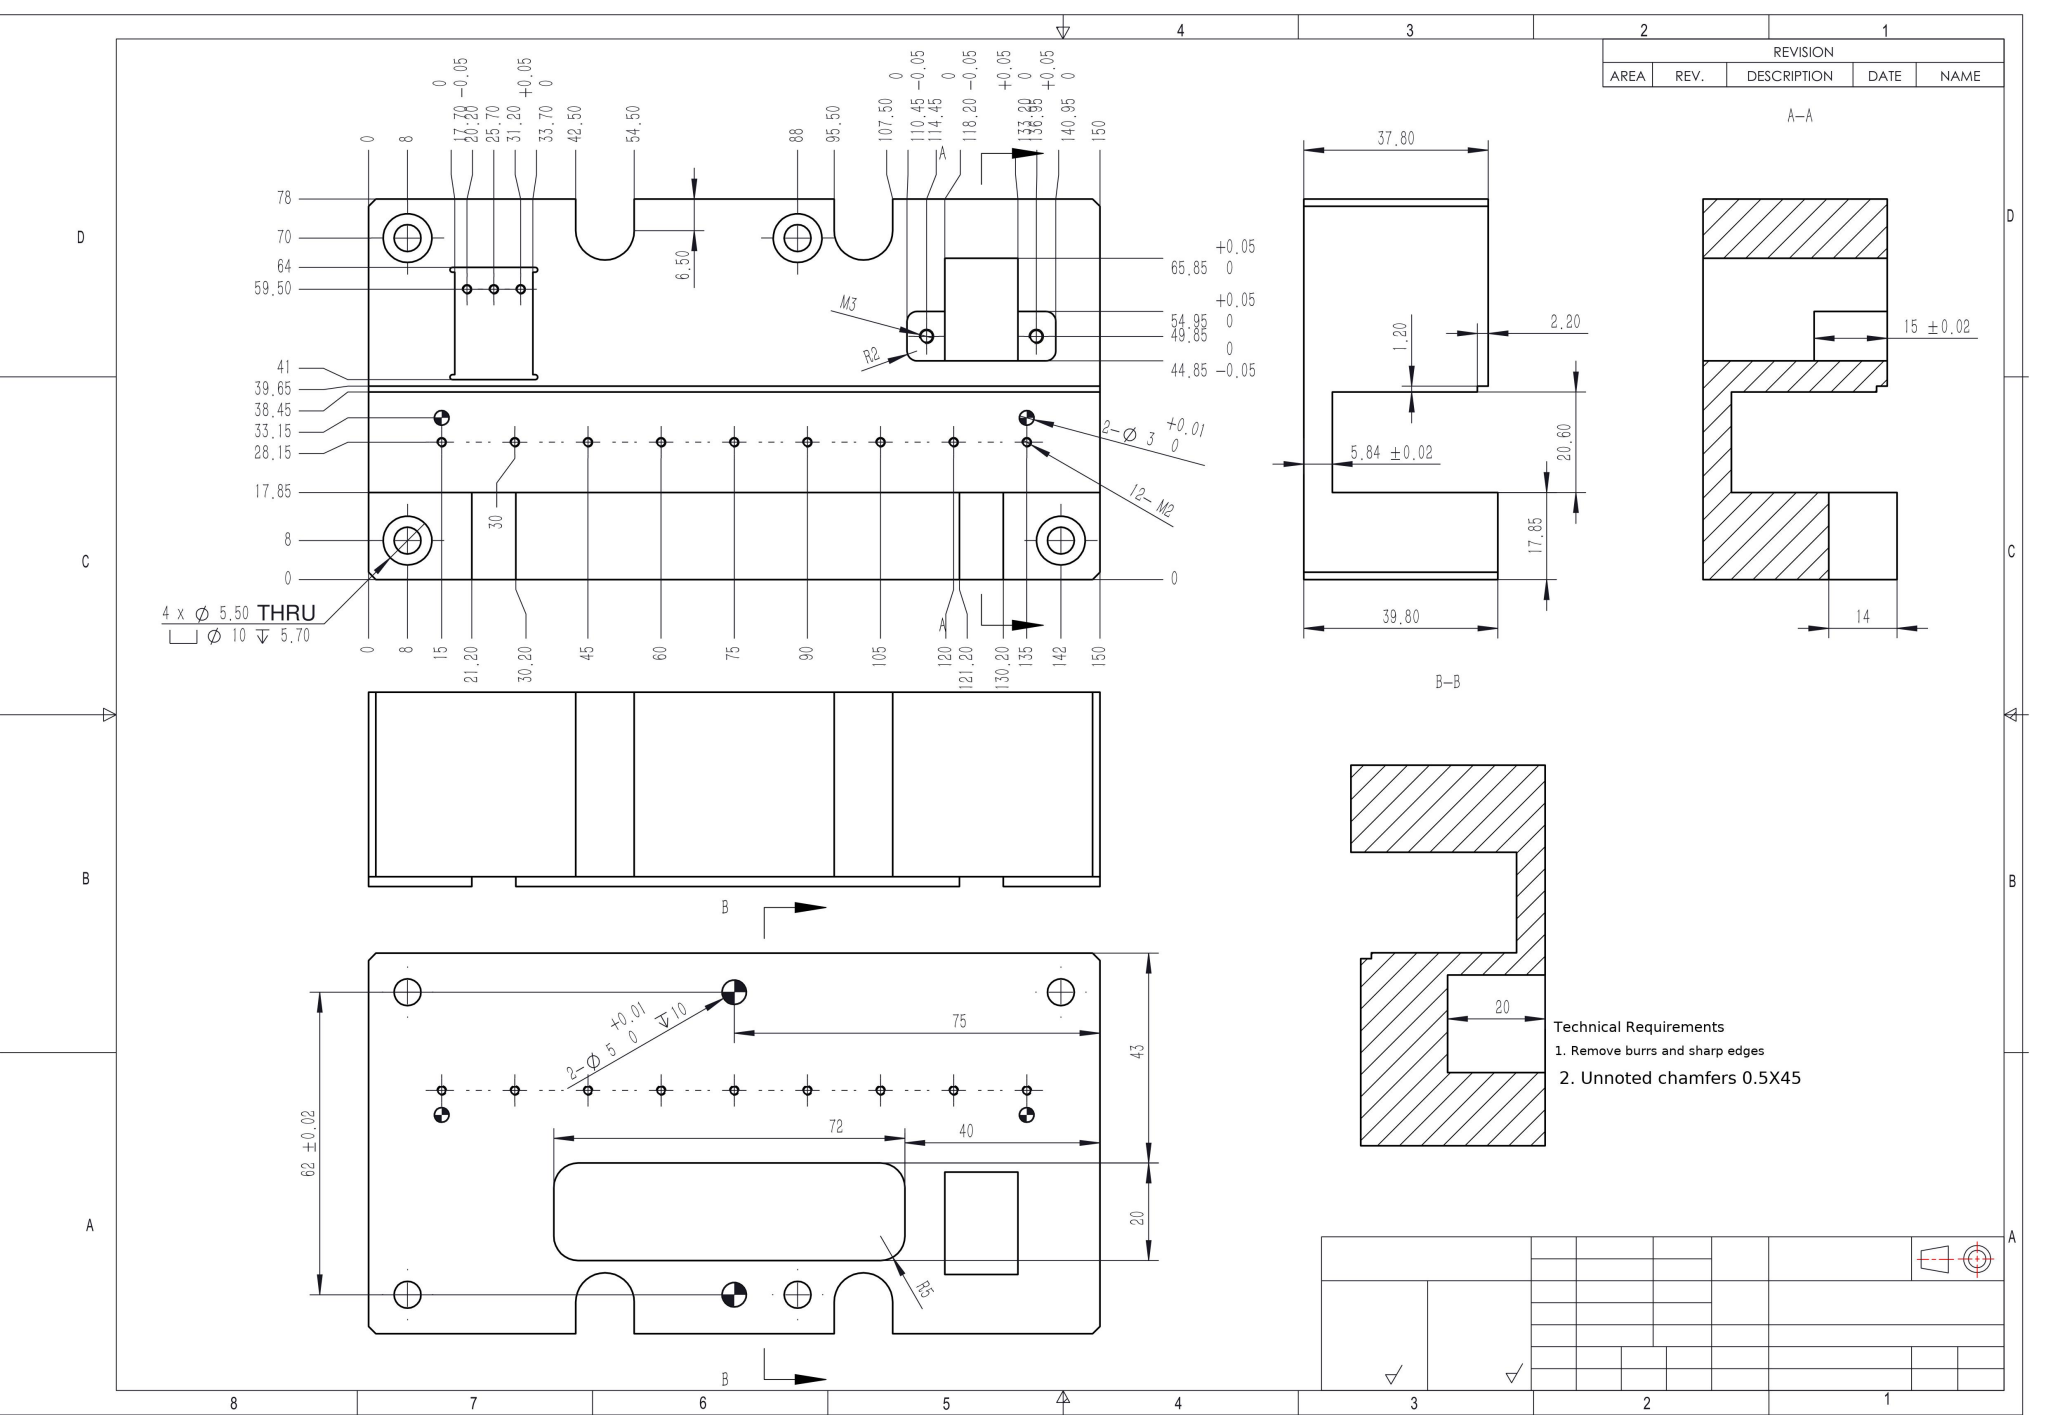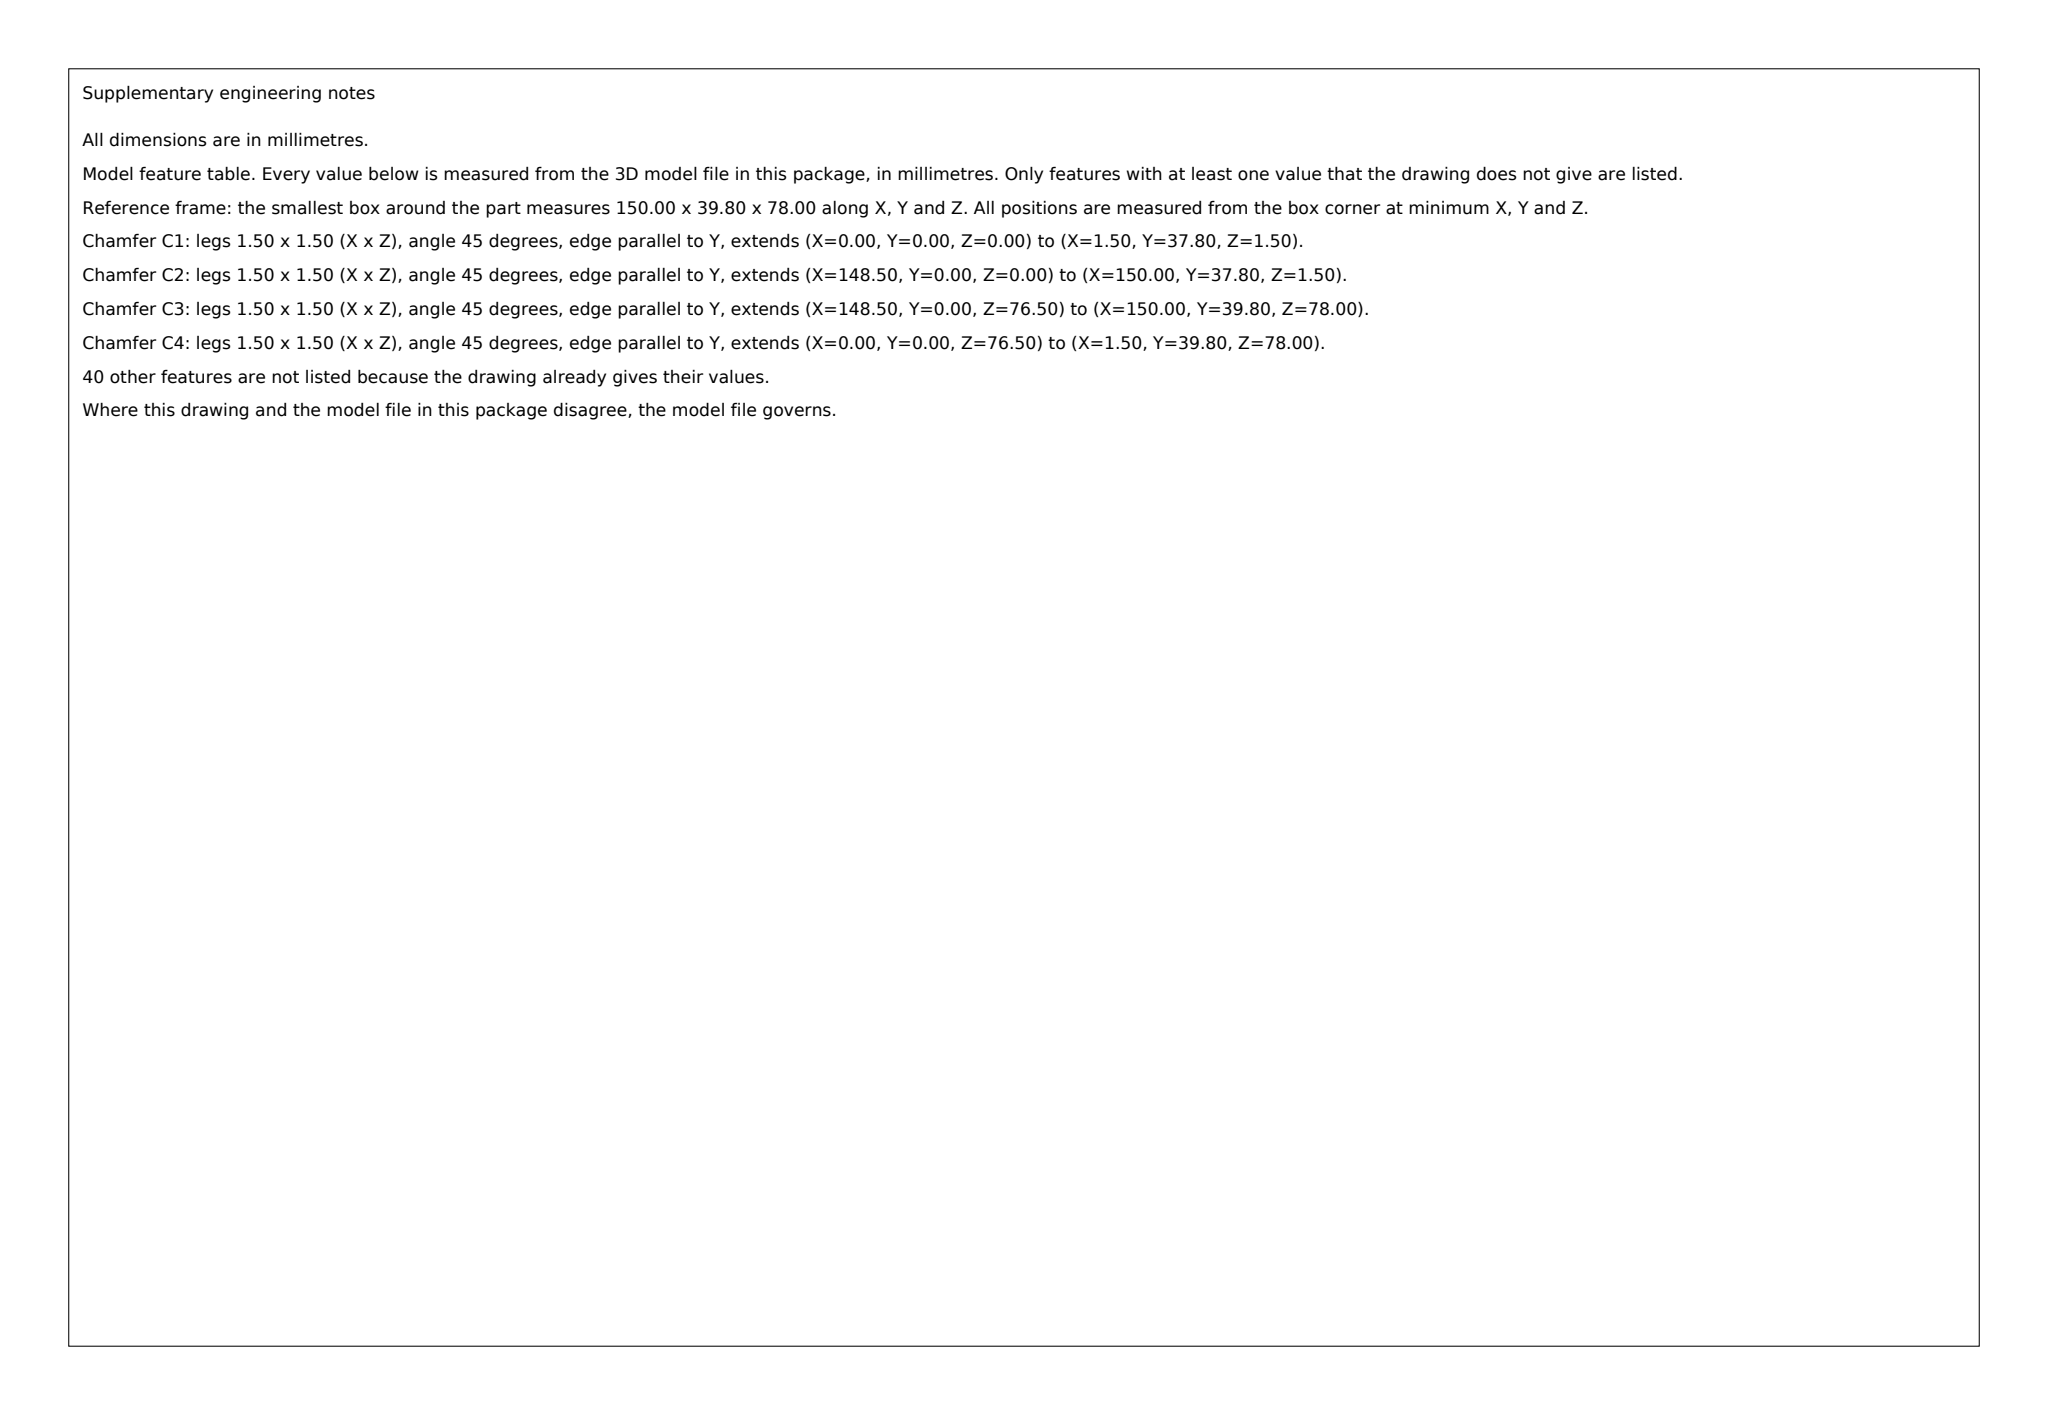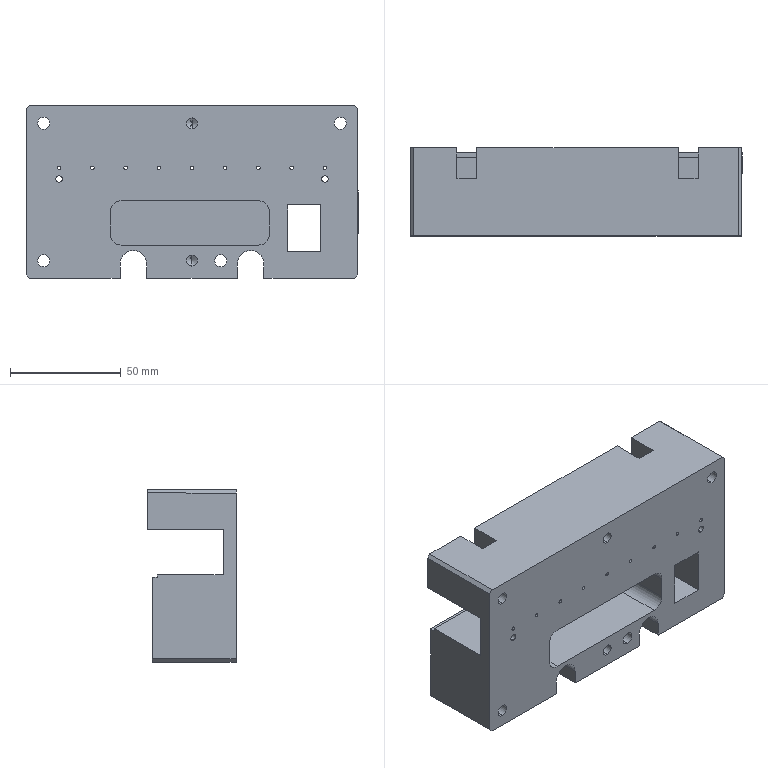Part | SolidWorks | mm | 1 solid | 140 faces | box 150 x 39.8 x 78 mm | volume 278440 mm3 | cylinder 68 | plane 58 | cone 14 | commonest cylinder face diameters 1.6 x24 10 x12 5.5 x8 2.5 x4 3 x4 5 x4 12 x4 4 x4